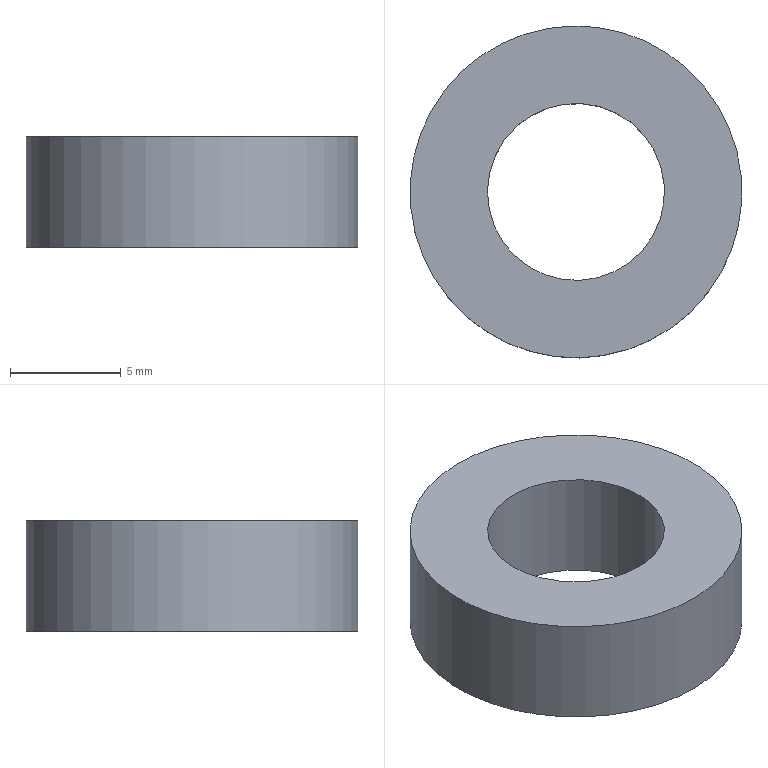Component | NX | FLANGE | 1 solid | 4 faces | box 15 x 15 x 5 mm | volume 632 mm3 | cylinder 2 | plane 2 | commonest cylinder face diameters 15 x1 8 x1
STEP:
#1=CARTESIAN_POINT('',(0.,0.,0.));
#2=DIRECTION('',(0.,0.,1.));
#3=DIRECTION('',(1.,0.,0.));
#4=AXIS2_PLACEMENT_3D('',#1,#2,#3);
#5=CARTESIAN_POINT('',(-200.883,-2.873,-2.));
#6=VERTEX_POINT('',#5);
#7=CARTESIAN_POINT('',(-193.955,0.,-2.));
#8=DIRECTION('',(0.,0.,-1.));
#9=DIRECTION('',(-0.9237,-0.383,0.));
#10=AXIS2_PLACEMENT_3D('',#7,#8,#9);
#11=CIRCLE('',#10,7.5);
#12=CARTESIAN_POINT('',(-193.955,0.,-2.));
#13=DIRECTION('',(0.,0.,1.));
#14=DIRECTION('',(0.9237,0.383,0.));
#15=AXIS2_PLACEMENT_3D('',#12,#13,#14);
#16=CYLINDRICAL_SURFACE('',#15,7.5);
#17=CARTESIAN_POINT('',(9.425,0.));
#18=DIRECTION('',(-1.,0.));
#19=VECTOR('',#18,1.);
#20=LINE('',#17,#19);
#21=(GEOMETRIC_REPRESENTATION_CONTEXT(2)PARAMETRIC_REPRESENTATION_CONTEXT()REPRESENTATION_CONTEXT('',''));
#22=DEFINITIONAL_REPRESENTATION('',(#20),#21);
#23=PCURVE('',#16,#22);
#24=CARTESIAN_POINT('',(-193.955,0.,-2.));
#25=DIRECTION('',(0.,0.,-1.));
#26=DIRECTION('',(-0.9237,-0.383,0.));
#27=AXIS2_PLACEMENT_3D('',#24,#25,#26);
#28=PLANE('',#27);
#29=CARTESIAN_POINT('',(0.,0.));
#30=DIRECTION('',(1.,-0.));
#31=AXIS2_PLACEMENT_2D('',#29,#30);
#32=CIRCLE('',#31,7.5);
#33=(GEOMETRIC_REPRESENTATION_CONTEXT(2)PARAMETRIC_REPRESENTATION_CONTEXT()REPRESENTATION_CONTEXT('',''));
#34=DEFINITIONAL_REPRESENTATION('',(#32),#33);
#35=PCURVE('',#28,#34);
#36=SURFACE_CURVE('',#11,(#23,#35),.PCURVE_S1.);
#37=EDGE_CURVE('',#6,#6,#36,.T.);
#38=ORIENTED_EDGE('',*,*,#37,.F.);
#39=CARTESIAN_POINT('',(-200.883,-2.873,3.));
#40=VERTEX_POINT('',#39);
#41=CARTESIAN_POINT('',(-200.883,-2.873,-2.));
#42=CARTESIAN_POINT('',(-200.883,-2.873,3.));
#43=B_SPLINE_CURVE_WITH_KNOTS('',1,(#41,#42),.UNSPECIFIED.,.F.,.F.,(2,2),(0.,5.),.PIECEWISE_BEZIER_KNOTS.);
#44=CARTESIAN_POINT('',(9.425,0.));
#45=DIRECTION('',(0.,1.));
#46=VECTOR('',#45,1.);
#47=LINE('',#44,#46);
#48=(GEOMETRIC_REPRESENTATION_CONTEXT(2)PARAMETRIC_REPRESENTATION_CONTEXT()REPRESENTATION_CONTEXT('',''));
#49=DEFINITIONAL_REPRESENTATION('',(#47),#48);
#50=PCURVE('',#16,#49);
#51=CARTESIAN_POINT('',(3.142,0.));
#52=DIRECTION('',(0.,1.));
#53=VECTOR('',#52,1.);
#54=LINE('',#51,#53);
#55=(GEOMETRIC_REPRESENTATION_CONTEXT(2)PARAMETRIC_REPRESENTATION_CONTEXT()REPRESENTATION_CONTEXT('',''));
#56=DEFINITIONAL_REPRESENTATION('',(#54),#55);
#57=PCURVE('',#16,#56);
#58=SEAM_CURVE('',#43,(#50,#57),.PCURVE_S1.);
#59=EDGE_CURVE('',#6,#40,#58,.T.);
#60=ORIENTED_EDGE('',*,*,#59,.T.);
#61=CARTESIAN_POINT('',(-193.955,0.,3.));
#62=DIRECTION('',(0.,0.,-1.));
#63=DIRECTION('',(-0.9237,-0.383,0.));
#64=AXIS2_PLACEMENT_3D('',#61,#62,#63);
#65=CIRCLE('',#64,7.5);
#66=CARTESIAN_POINT('',(9.425,5.));
#67=DIRECTION('',(-1.,0.));
#68=VECTOR('',#67,1.);
#69=LINE('',#66,#68);
#70=(GEOMETRIC_REPRESENTATION_CONTEXT(2)PARAMETRIC_REPRESENTATION_CONTEXT()REPRESENTATION_CONTEXT('',''));
#71=DEFINITIONAL_REPRESENTATION('',(#69),#70);
#72=PCURVE('',#16,#71);
#73=CARTESIAN_POINT('',(-193.955,0.,3.));
#74=DIRECTION('',(0.,0.,-1.));
#75=DIRECTION('',(-0.9237,-0.383,0.));
#76=AXIS2_PLACEMENT_3D('',#73,#74,#75);
#77=PLANE('',#76);
#78=CARTESIAN_POINT('',(0.,0.));
#79=DIRECTION('',(1.,-0.));
#80=AXIS2_PLACEMENT_2D('',#78,#79);
#81=CIRCLE('',#80,7.5);
#82=(GEOMETRIC_REPRESENTATION_CONTEXT(2)PARAMETRIC_REPRESENTATION_CONTEXT()REPRESENTATION_CONTEXT('',''));
#83=DEFINITIONAL_REPRESENTATION('',(#81),#82);
#84=PCURVE('',#77,#83);
#85=SURFACE_CURVE('',#65,(#72,#84),.PCURVE_S1.);
#86=EDGE_CURVE('',#40,#40,#85,.T.);
#87=ORIENTED_EDGE('',*,*,#86,.T.);
#88=ORIENTED_EDGE('',*,*,#59,.F.);
#89=EDGE_LOOP('',(#38,#60,#87,#88));
#90=FACE_BOUND('',#89,.T.);
#91=ADVANCED_FACE('',(#90),#16,.T.);
#92=CARTESIAN_POINT('',(-197.65,-1.532,-2.));
#93=VERTEX_POINT('',#92);
#94=CARTESIAN_POINT('',(-193.955,0.,-2.));
#95=DIRECTION('',(0.,0.,-1.));
#96=DIRECTION('',(-0.9237,-0.383,0.));
#97=AXIS2_PLACEMENT_3D('',#94,#95,#96);
#98=CIRCLE('',#97,4.);
#99=CARTESIAN_POINT('',(-193.955,0.,-2.));
#100=DIRECTION('',(0.,0.,1.));
#101=DIRECTION('',(0.9237,0.383,0.));
#102=AXIS2_PLACEMENT_3D('',#99,#100,#101);
#103=CYLINDRICAL_SURFACE('',#102,4.);
#104=CARTESIAN_POINT('',(9.425,0.));
#105=DIRECTION('',(-1.,0.));
#106=VECTOR('',#105,1.);
#107=LINE('',#104,#106);
#108=(GEOMETRIC_REPRESENTATION_CONTEXT(2)PARAMETRIC_REPRESENTATION_CONTEXT()REPRESENTATION_CONTEXT('',''));
#109=DEFINITIONAL_REPRESENTATION('',(#107),#108);
#110=PCURVE('',#103,#109);
#111=CARTESIAN_POINT('',(0.,0.));
#112=DIRECTION('',(1.,0.));
#113=AXIS2_PLACEMENT_2D('',#111,#112);
#114=CIRCLE('',#113,4.);
#115=(GEOMETRIC_REPRESENTATION_CONTEXT(2)PARAMETRIC_REPRESENTATION_CONTEXT()REPRESENTATION_CONTEXT('',''));
#116=DEFINITIONAL_REPRESENTATION('',(#114),#115);
#117=PCURVE('',#28,#116);
#118=SURFACE_CURVE('',#98,(#110,#117),.PCURVE_S1.);
#119=EDGE_CURVE('',#93,#93,#118,.T.);
#120=ORIENTED_EDGE('',*,*,#119,.F.);
#121=CARTESIAN_POINT('',(-197.65,-1.532,3.));
#122=VERTEX_POINT('',#121);
#123=CARTESIAN_POINT('',(-197.65,-1.532,-2.));
#124=CARTESIAN_POINT('',(-197.65,-1.532,3.));
#125=B_SPLINE_CURVE_WITH_KNOTS('',1,(#123,#124),.UNSPECIFIED.,.F.,.F.,(2,2),(0.,5.),.PIECEWISE_BEZIER_KNOTS.);
#126=CARTESIAN_POINT('',(9.425,0.));
#127=DIRECTION('',(0.,1.));
#128=VECTOR('',#127,1.);
#129=LINE('',#126,#128);
#130=(GEOMETRIC_REPRESENTATION_CONTEXT(2)PARAMETRIC_REPRESENTATION_CONTEXT()REPRESENTATION_CONTEXT('',''));
#131=DEFINITIONAL_REPRESENTATION('',(#129),#130);
#132=PCURVE('',#103,#131);
#133=CARTESIAN_POINT('',(3.142,0.));
#134=DIRECTION('',(0.,1.));
#135=VECTOR('',#134,1.);
#136=LINE('',#133,#135);
#137=(GEOMETRIC_REPRESENTATION_CONTEXT(2)PARAMETRIC_REPRESENTATION_CONTEXT()REPRESENTATION_CONTEXT('',''));
#138=DEFINITIONAL_REPRESENTATION('',(#136),#137);
#139=PCURVE('',#103,#138);
#140=SEAM_CURVE('',#125,(#132,#139),.PCURVE_S1.);
#141=EDGE_CURVE('',#93,#122,#140,.T.);
#142=ORIENTED_EDGE('',*,*,#141,.T.);
#143=CARTESIAN_POINT('',(-193.955,0.,3.));
#144=DIRECTION('',(0.,0.,-1.));
#145=DIRECTION('',(-0.9237,-0.383,0.));
#146=AXIS2_PLACEMENT_3D('',#143,#144,#145);
#147=CIRCLE('',#146,4.);
#148=CARTESIAN_POINT('',(9.425,5.));
#149=DIRECTION('',(-1.,0.));
#150=VECTOR('',#149,1.);
#151=LINE('',#148,#150);
#152=(GEOMETRIC_REPRESENTATION_CONTEXT(2)PARAMETRIC_REPRESENTATION_CONTEXT()REPRESENTATION_CONTEXT('',''));
#153=DEFINITIONAL_REPRESENTATION('',(#151),#152);
#154=PCURVE('',#103,#153);
#155=CARTESIAN_POINT('',(0.,0.));
#156=DIRECTION('',(1.,0.));
#157=AXIS2_PLACEMENT_2D('',#155,#156);
#158=CIRCLE('',#157,4.);
#159=(GEOMETRIC_REPRESENTATION_CONTEXT(2)PARAMETRIC_REPRESENTATION_CONTEXT()REPRESENTATION_CONTEXT('',''));
#160=DEFINITIONAL_REPRESENTATION('',(#158),#159);
#161=PCURVE('',#77,#160);
#162=SURFACE_CURVE('',#147,(#154,#161),.PCURVE_S1.);
#163=EDGE_CURVE('',#122,#122,#162,.T.);
#164=ORIENTED_EDGE('',*,*,#163,.T.);
#165=ORIENTED_EDGE('',*,*,#141,.F.);
#166=EDGE_LOOP('',(#120,#142,#164,#165));
#167=FACE_BOUND('',#166,.F.);
#168=ADVANCED_FACE('',(#167),#103,.F.);
#169=ORIENTED_EDGE('',*,*,#37,.T.);
#170=EDGE_LOOP('',(#169));
#171=FACE_BOUND('',#170,.T.);
#172=ORIENTED_EDGE('',*,*,#119,.F.);
#173=EDGE_LOOP('',(#172));
#174=FACE_BOUND('',#173,.T.);
#175=ADVANCED_FACE('',(#171,#174),#28,.T.);
#176=ORIENTED_EDGE('',*,*,#86,.F.);
#177=EDGE_LOOP('',(#176));
#178=FACE_BOUND('',#177,.T.);
#179=ORIENTED_EDGE('',*,*,#163,.T.);
#180=EDGE_LOOP('',(#179));
#181=FACE_BOUND('',#180,.T.);
#182=ADVANCED_FACE('',(#178,#181),#77,.F.);
#183=CLOSED_SHELL('',(#91,#168,#175,#182));
#184=MANIFOLD_SOLID_BREP('',#183);
#185=(LENGTH_UNIT()NAMED_UNIT(*)SI_UNIT(.MILLI.,.METRE.));
#186=UNCERTAINTY_MEASURE_WITH_UNIT(LENGTH_MEASURE(0.00001),#185,'','');
#187=(NAMED_UNIT(*)PLANE_ANGLE_UNIT()SI_UNIT($,.RADIAN.));
#188=(NAMED_UNIT(*)SI_UNIT($,.STERADIAN.)SOLID_ANGLE_UNIT());
#189=(GEOMETRIC_REPRESENTATION_CONTEXT(3)GLOBAL_UNCERTAINTY_ASSIGNED_CONTEXT((#186))GLOBAL_UNIT_ASSIGNED_CONTEXT((#185,#187,#188))REPRESENTATION_CONTEXT('',''));
#190=ADVANCED_BREP_SHAPE_REPRESENTATION('',(#4,#184),#189);